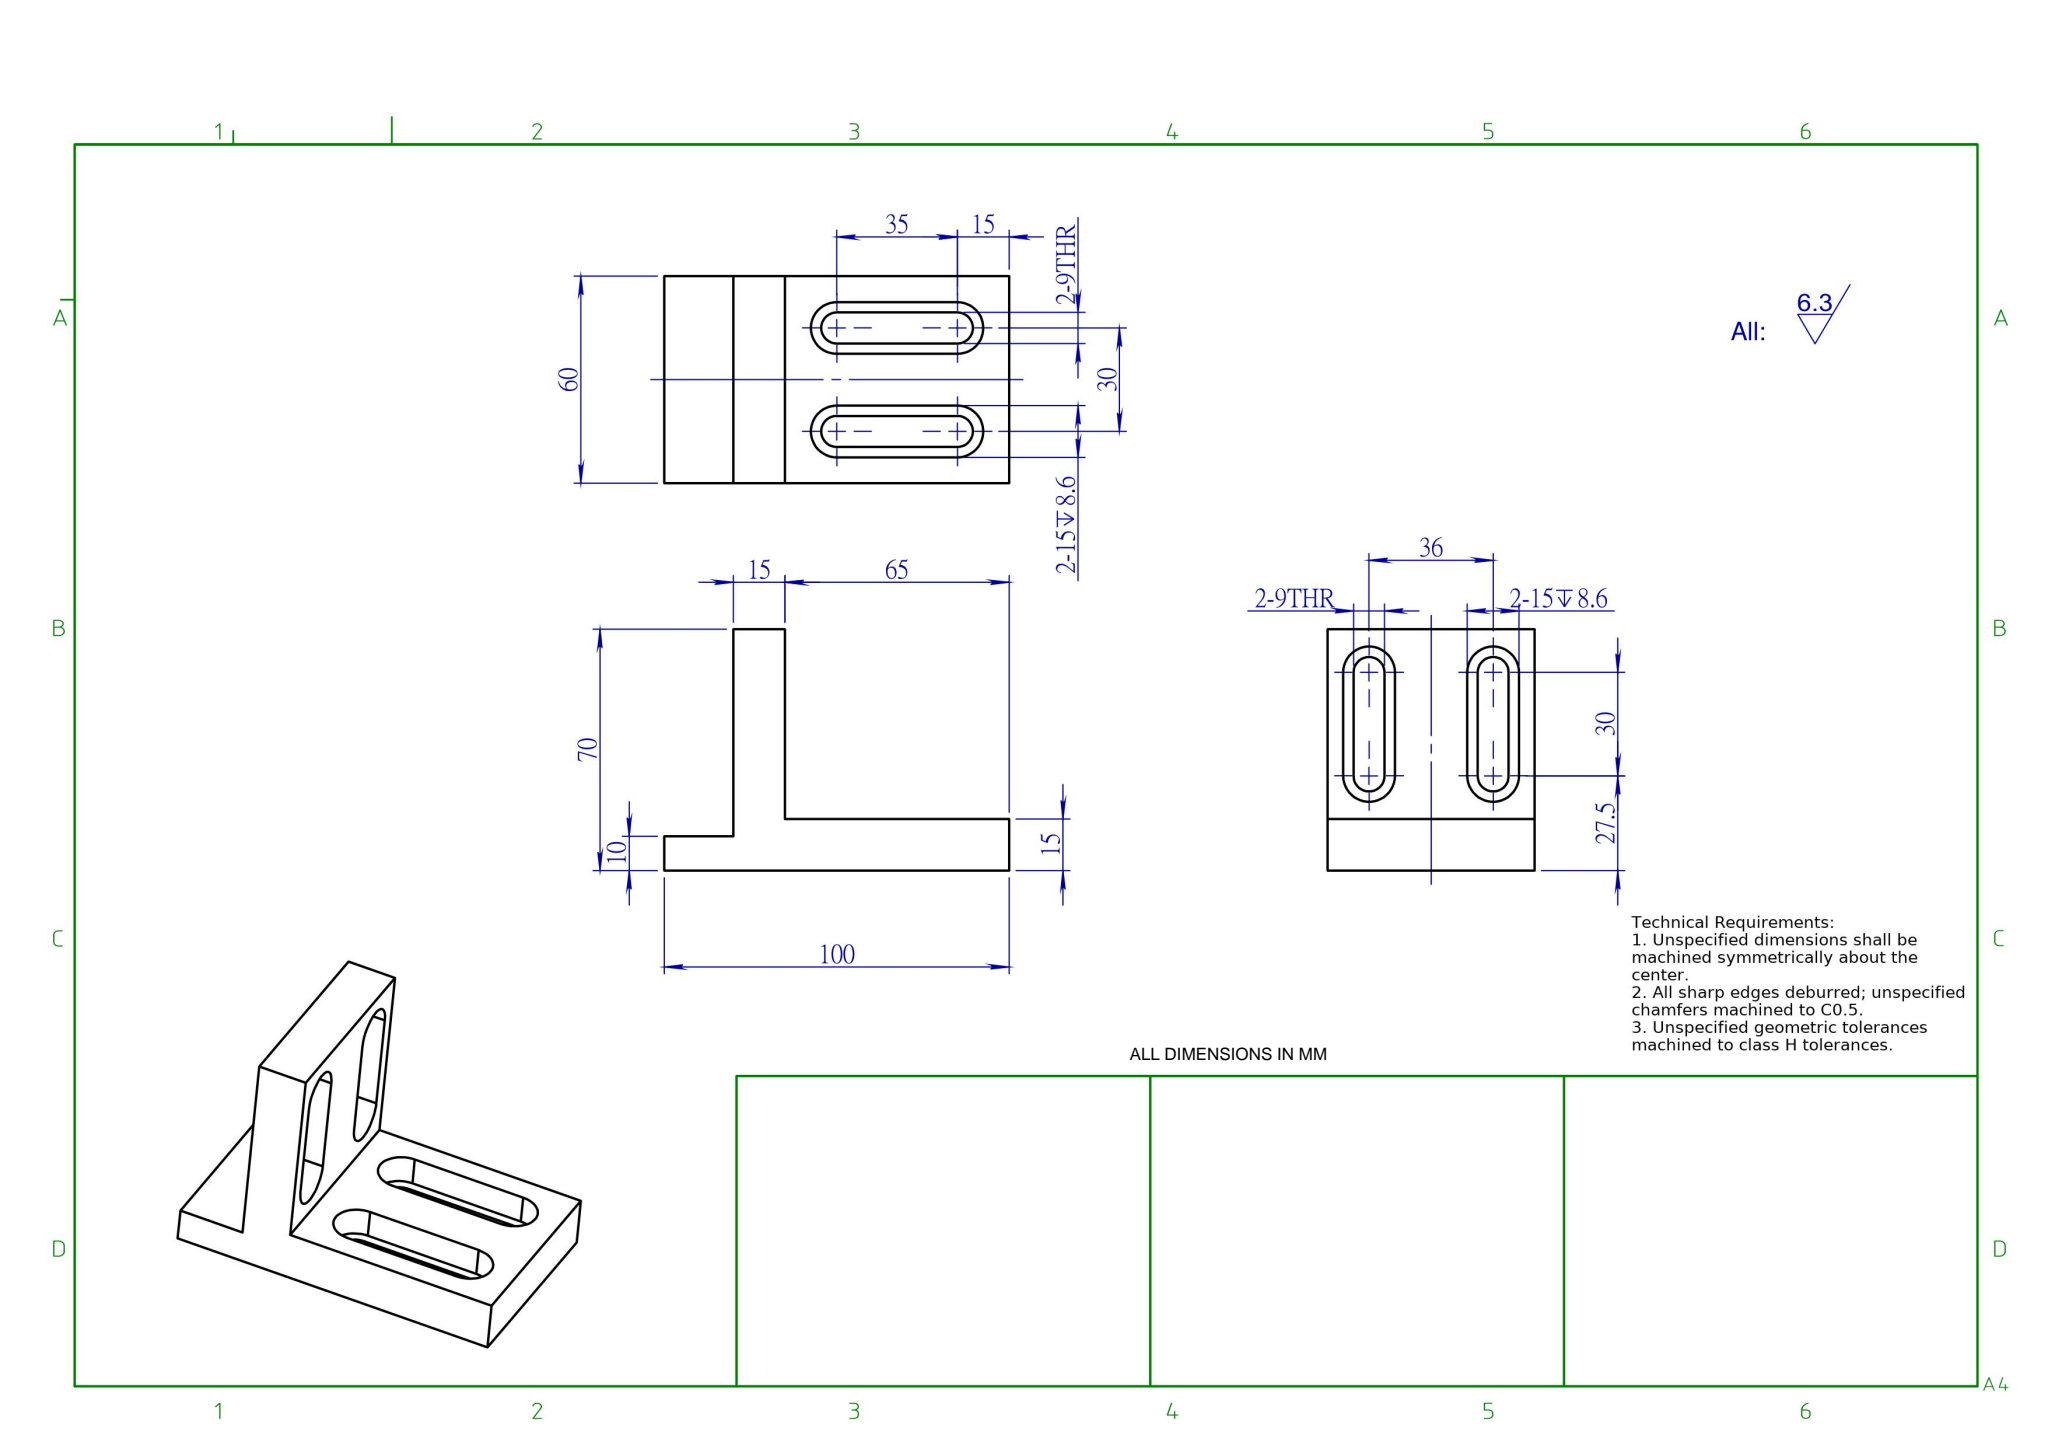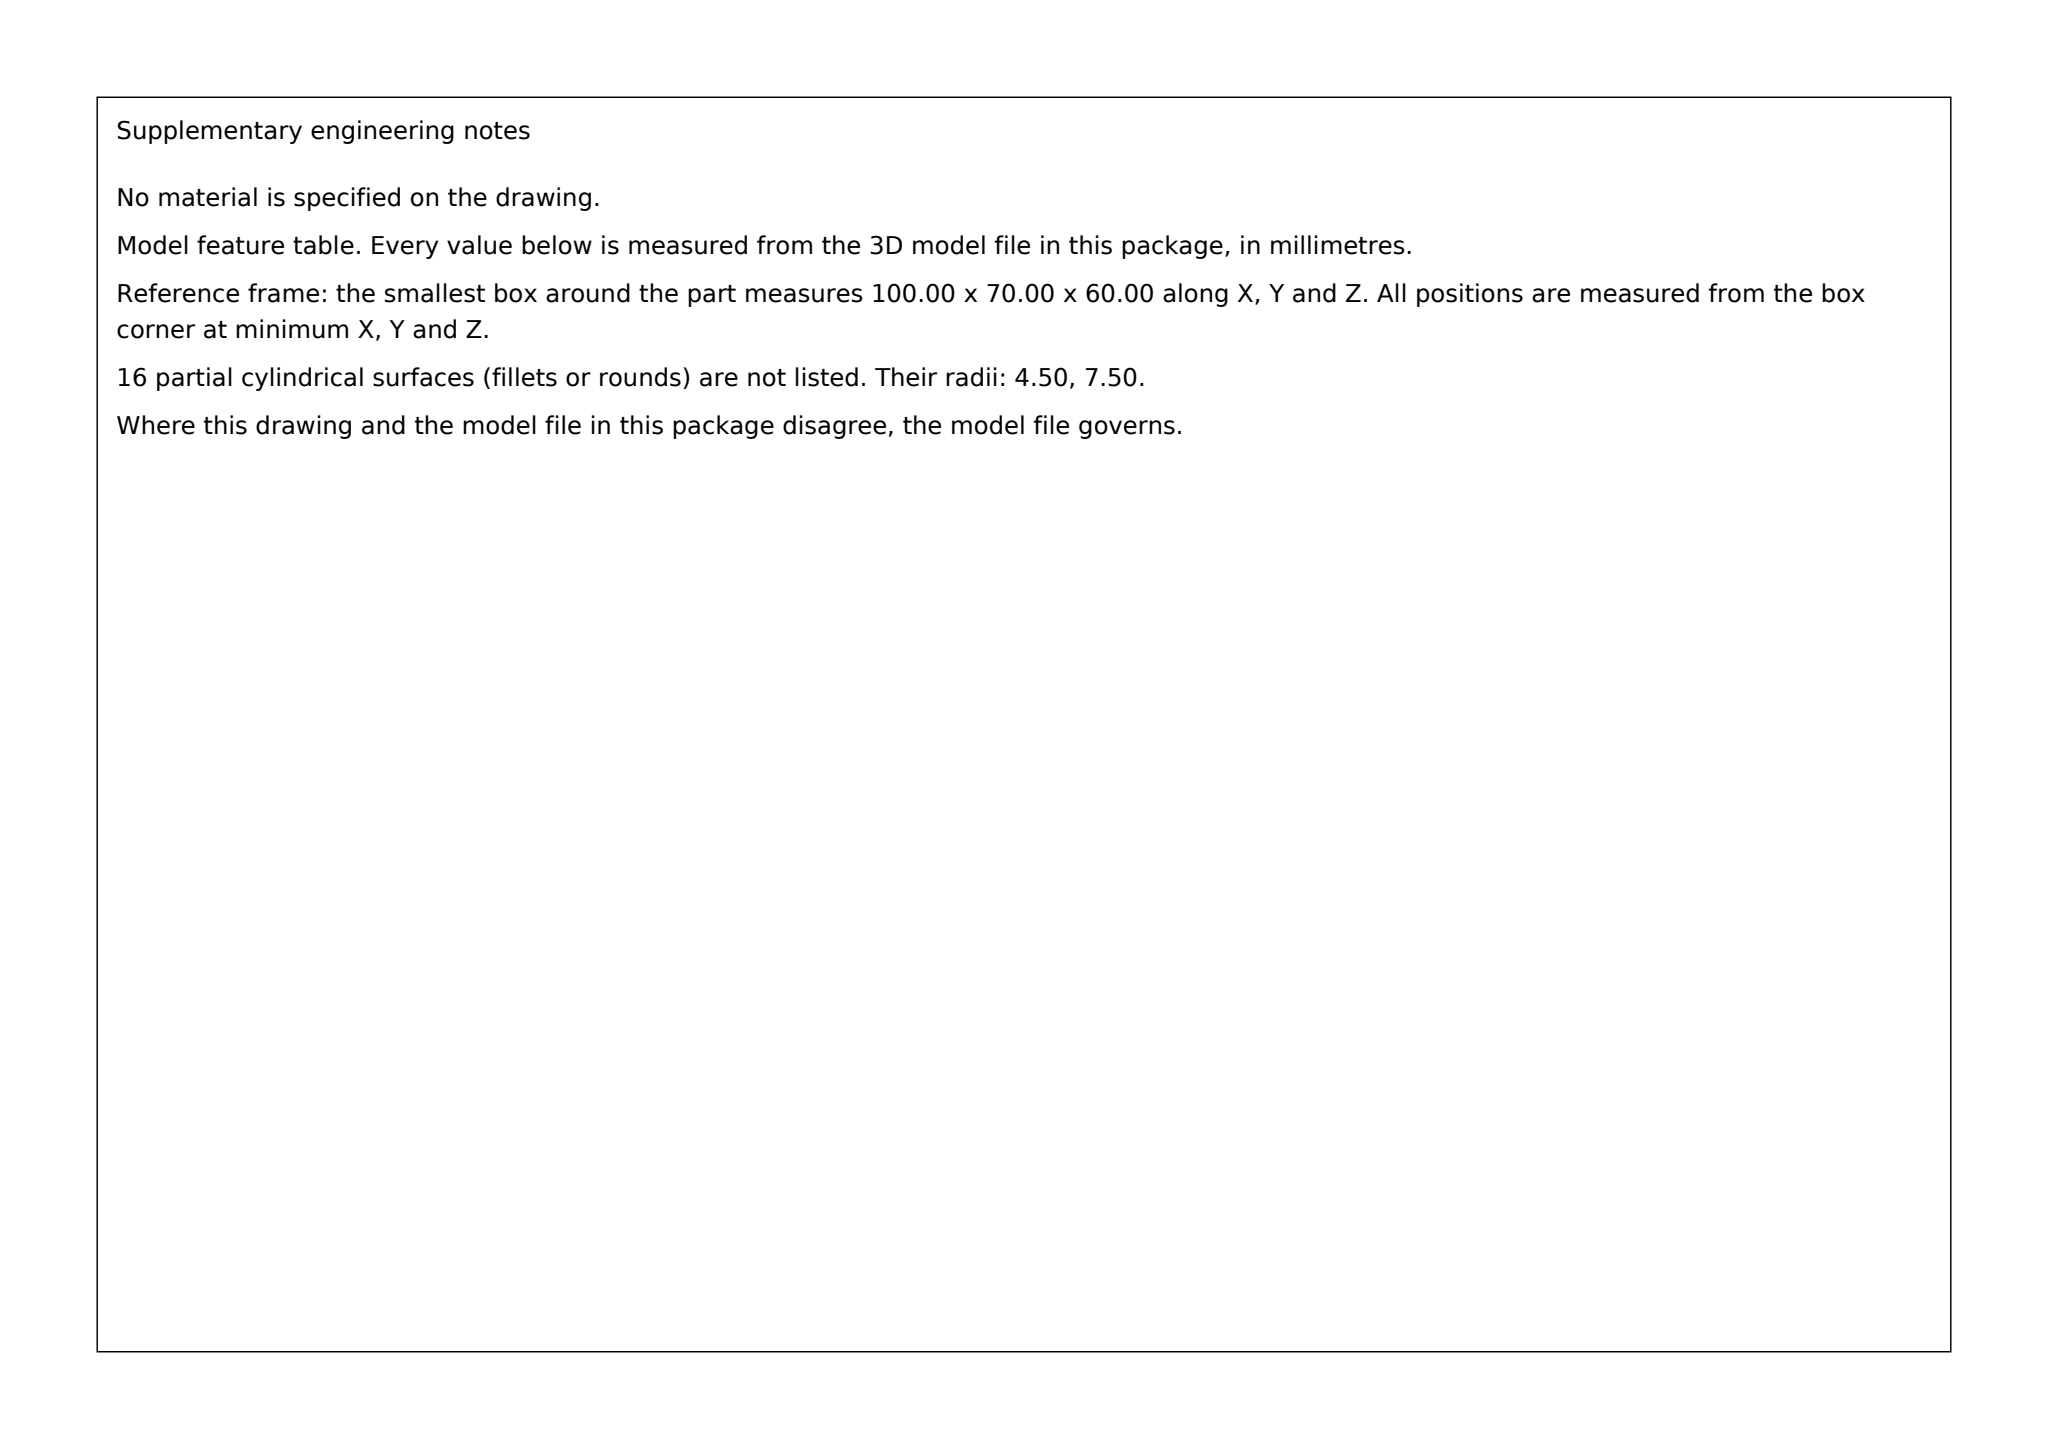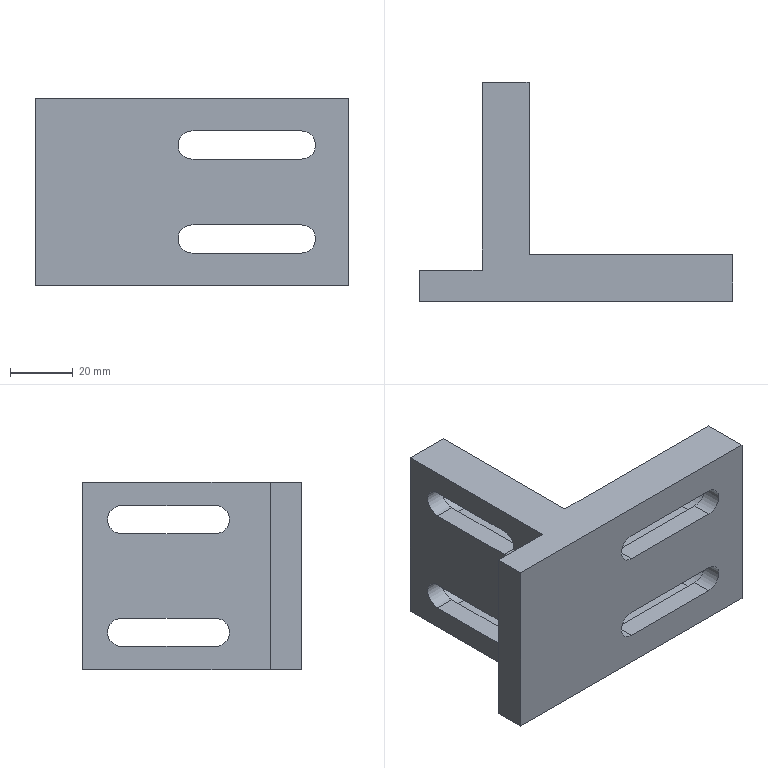Part | SolidWorks | mm | 1 solid | 46 faces | box 100 x 70 x 60 mm | volume 101534 mm3 | plane 30 | cylinder 16 | commonest cylinder face diameters 9 x8 15 x8
build123d program:
from build123d import *

# Parameters (mm, degrees)
SKETCH1_W           = 80
SKETCH1_H           = 15
BOSS_EXTRUDE1_DEPTH = 30
SKETCH2_W           = 15
SKETCH2_H           = 60
BOSS_EXTRUDE2_DEPTH = 55
CUT_EXTRUDE1_DEPTH  = 102.612
CUT_EXTRUDE3_DEPTH  = 8.6
CUT_EXTRUDE4_DEPTH  = 8.6
CUT_EXTRUDE5_DEPTH  = 97.654
SKETCH11_W          = 60
SKETCH11_H          = 10
BOSS_EXTRUDE3_DEPTH = 20


with BuildPart() as part:
    # Sketch1 → Boss-Extrude1 (new, symmetric)
    with BuildSketch(Plane.XY):
        with Locations((40, -7.5)):
            Rectangle(SKETCH1_W, SKETCH1_H)
    extrude(amount=BOSS_EXTRUDE1_DEPTH, both=True)

    # Sketch2 → Boss-Extrude2 (add)
    with BuildSketch(Plane(origin=(0, 0, 0), x_dir=(1, 0, 0), z_dir=(0, 1, 0))):
        with Locations((7.5, 0)):
            Rectangle(SKETCH2_W, SKETCH2_H)
    extrude(amount=BOSS_EXTRUDE2_DEPTH)

    # Sketch3 → Cut-Extrude1 (cut, through all)
    with BuildSketch(Plane(origin=(0, 0, 0), x_dir=(1, 0, 0), z_dir=(0, 1, 0))):
        with BuildLine():
            Line((30, 19.5), (65, 19.5))
            ThreePointArc((65, 19.5), (69.5, 15), (65, 10.5))
            Line((65, 10.5), (30, 10.5))
            ThreePointArc((30, 10.5), (25.5, 15), (30, 19.5))
        make_face()
        with BuildLine():
            Line((30, -19.5), (65, -19.5))
            ThreePointArc((65, -19.5), (69.5, -15), (65, -10.5))
            Line((65, -10.5), (30, -10.5))
            ThreePointArc((30, -10.5), (25.5, -15), (30, -19.5))
        make_face()
    extrude(amount=-CUT_EXTRUDE1_DEPTH, mode=Mode.SUBTRACT)

    # Sketch7 → Cut-Extrude3 (cut)
    with BuildSketch(Plane(origin=(0, 0, 0), x_dir=(1, 0, 0), z_dir=(0, 1, 0))):
        with BuildLine():
            Line((30, 22.5), (65, 22.5))
            ThreePointArc((65, 22.5), (72.5, 15), (65, 7.5))
            Line((65, 7.5), (30, 7.5))
            ThreePointArc((30, 7.5), (22.5, 15), (30, 22.5))
        make_face()
        with BuildLine():
            Line((30, -7.5), (65, -7.5))
            ThreePointArc((65, -7.5), (72.5, -15), (65, -22.5))
            Line((65, -22.5), (30, -22.5))
            ThreePointArc((30, -22.5), (22.5, -15), (30, -7.5))
        make_face()
    extrude(amount=-CUT_EXTRUDE3_DEPTH, mode=Mode.SUBTRACT)

    # Sketch8 → Cut-Extrude4 (cut)
    with BuildSketch(Plane(origin=(15, 0, 0), x_dir=(0, 0, -1), z_dir=(1, 0, 0))):
        with BuildLine():
            Line((-10.5, 42.5), (-10.5, 12.5))
            ThreePointArc((-10.5, 12.5), (-18, 5), (-25.5, 12.5))
            Line((-25.5, 12.5), (-25.5, 42.5))
            ThreePointArc((-25.5, 42.5), (-18, 50), (-10.5, 42.5))
        make_face()
        with BuildLine():
            Line((25.5, 42.5), (25.5, 12.5))
            ThreePointArc((25.5, 12.5), (18, 5), (10.5, 12.5))
            Line((10.5, 12.5), (10.5, 42.5))
            ThreePointArc((10.5, 42.5), (18, 50), (25.5, 42.5))
        make_face()
    extrude(amount=-CUT_EXTRUDE4_DEPTH, mode=Mode.SUBTRACT)

    # Sketch9 → Cut-Extrude5 (cut, through all)
    with BuildSketch(Plane(origin=(6.4, 0, 0), x_dir=(0, 0, -1), z_dir=(1, 0, 0))):
        with BuildLine():
            Line((-22.5, 42.5), (-22.5, 12.5))
            ThreePointArc((-22.5, 12.5), (-18, 8), (-13.5, 12.5))
            Line((-13.5, 12.5), (-13.5, 42.5))
            ThreePointArc((-13.5, 42.5), (-18, 47), (-22.5, 42.5))
        make_face()
        with BuildLine():
            Line((13.5, 42.5), (13.5, 12.5))
            ThreePointArc((13.5, 12.5), (18, 8), (22.5, 12.5))
            Line((22.5, 12.5), (22.5, 42.5))
            ThreePointArc((22.5, 42.5), (18, 47), (13.5, 42.5))
        make_face()
    extrude(amount=-CUT_EXTRUDE5_DEPTH, mode=Mode.SUBTRACT)

    # Sketch11 → Boss-Extrude3 (add)
    with BuildSketch(Plane.ZY):
        with Locations((0, -10)):
            Rectangle(SKETCH11_W, SKETCH11_H)
    extrude(amount=BOSS_EXTRUDE3_DEPTH)


solid = part.part